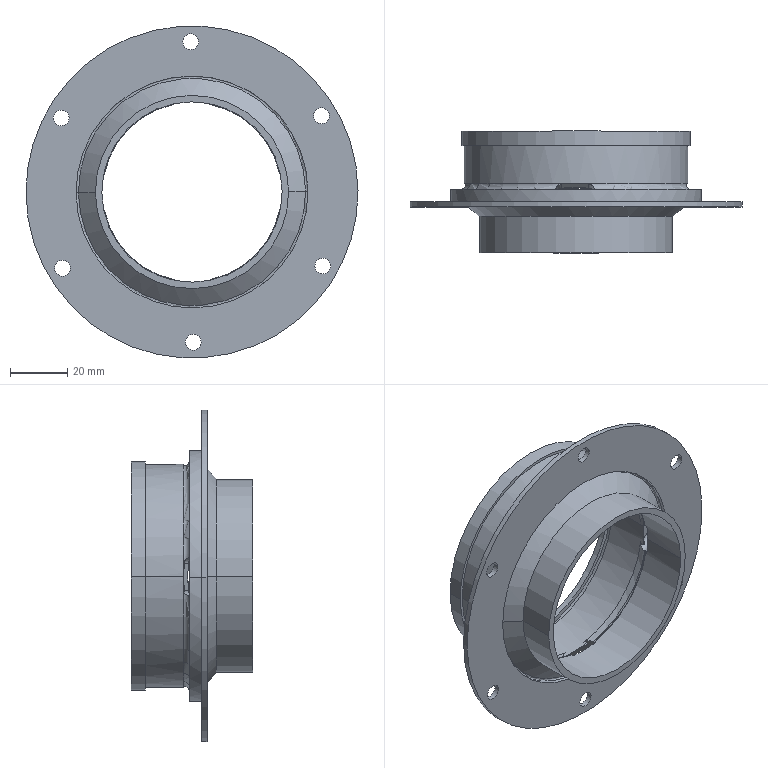Component | SolidWorks | TurbineBearingHousing-1 | 1 solid | 99 faces | volume 45163 mm3 | cylinder 44 | plane 39 | torus 14 | cone 2 | commonest cylinder face diameters 5.5 x12 3.8 x8 72 x4 66.5 x4 75 x2 80 x2 116 x2 81 x2